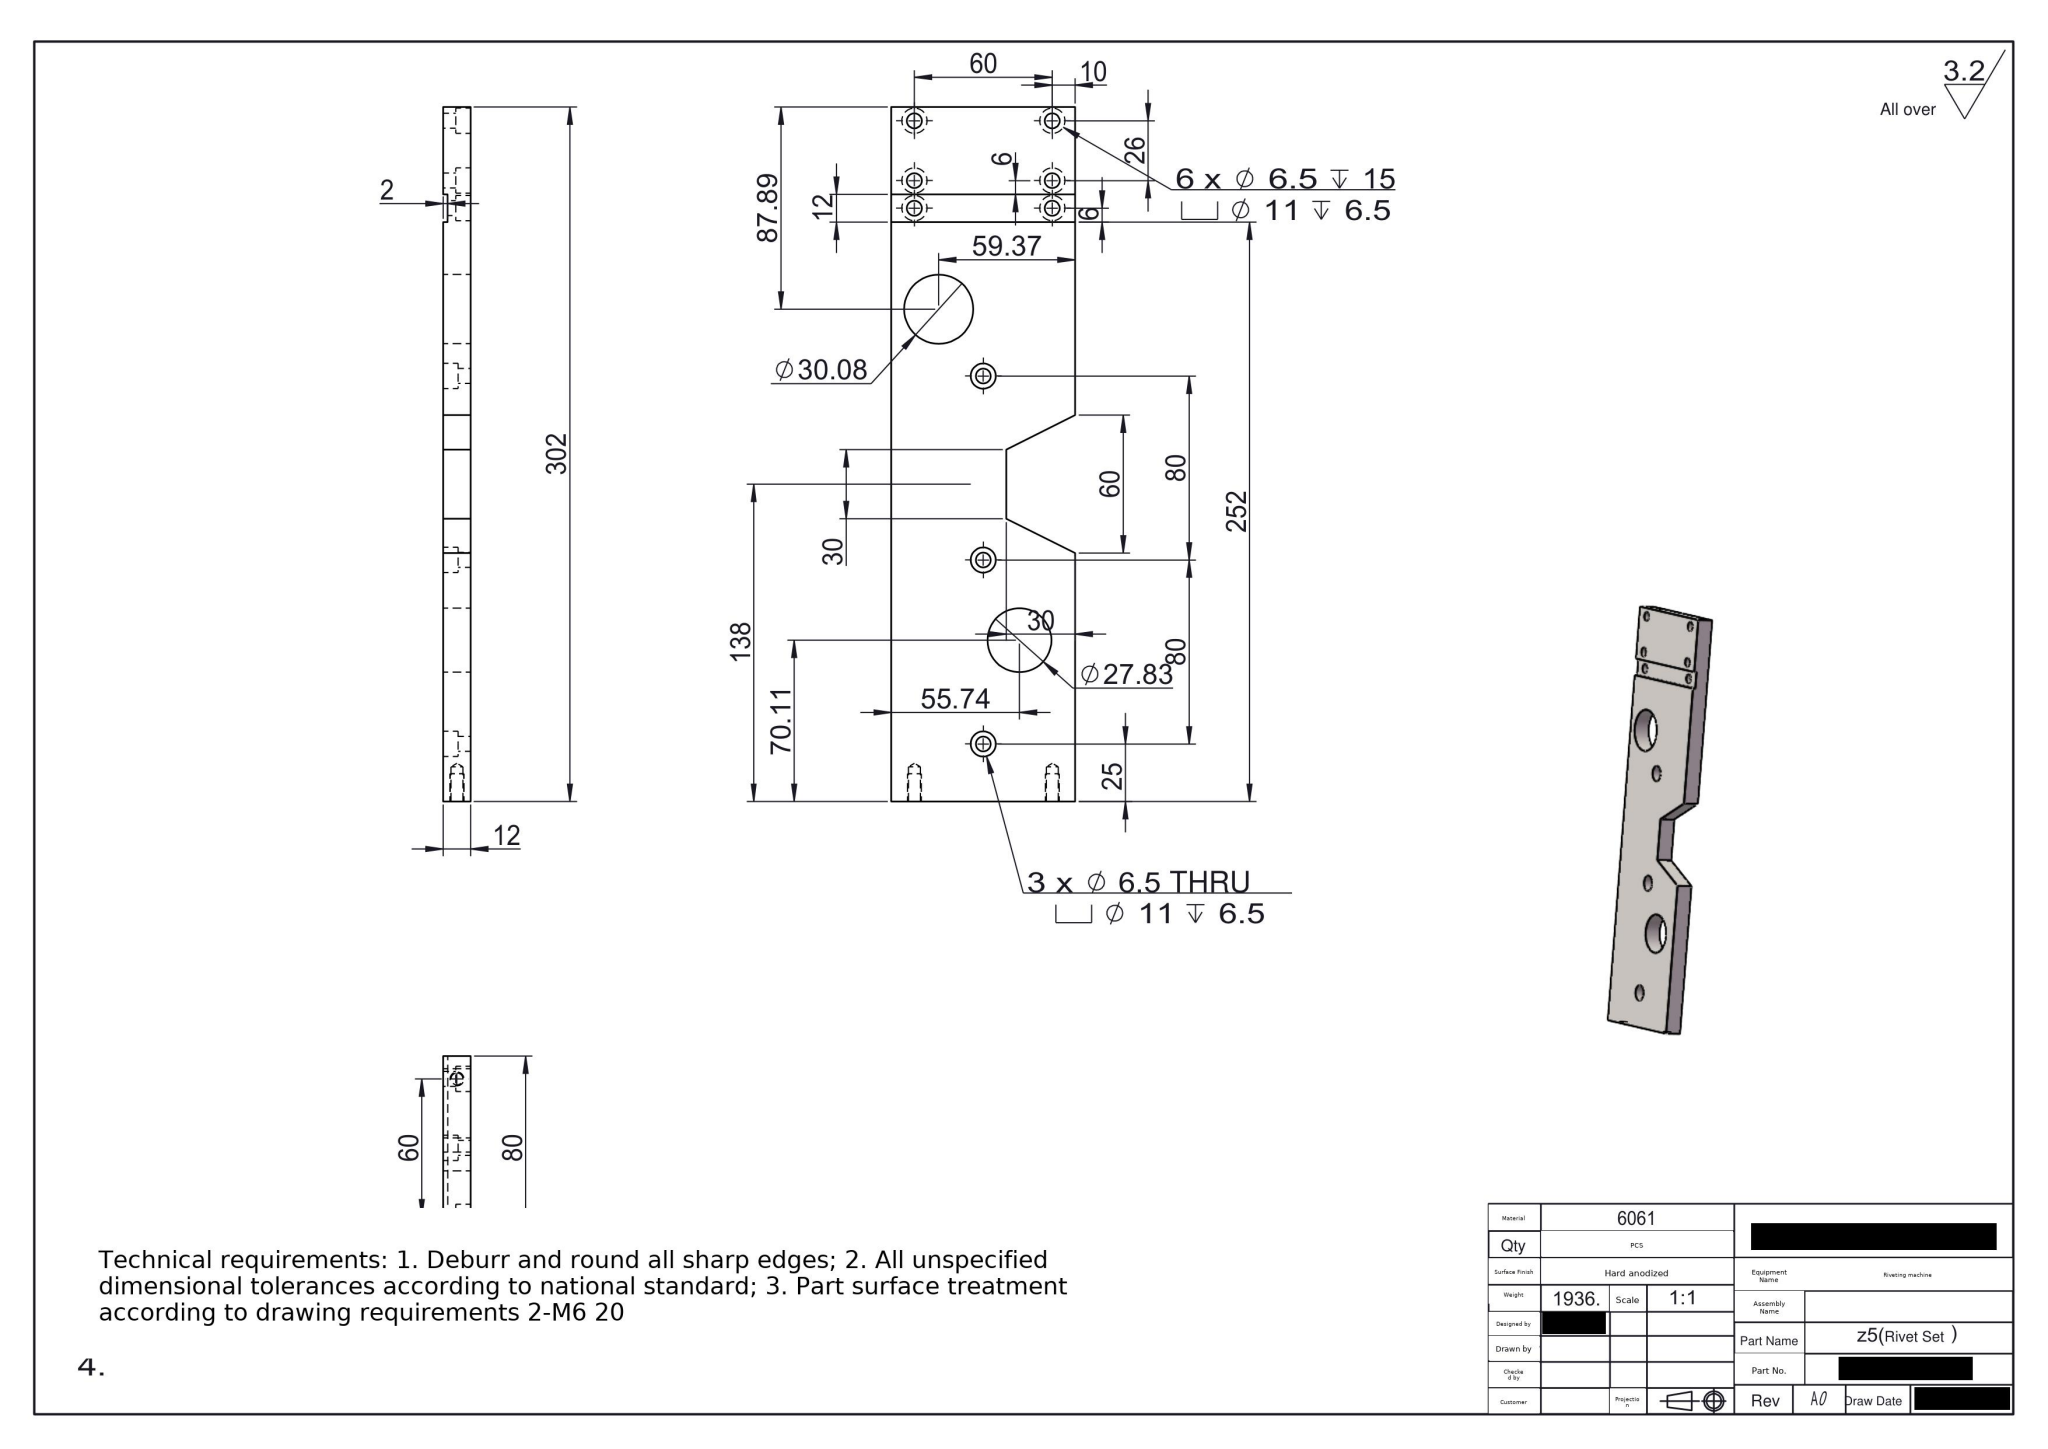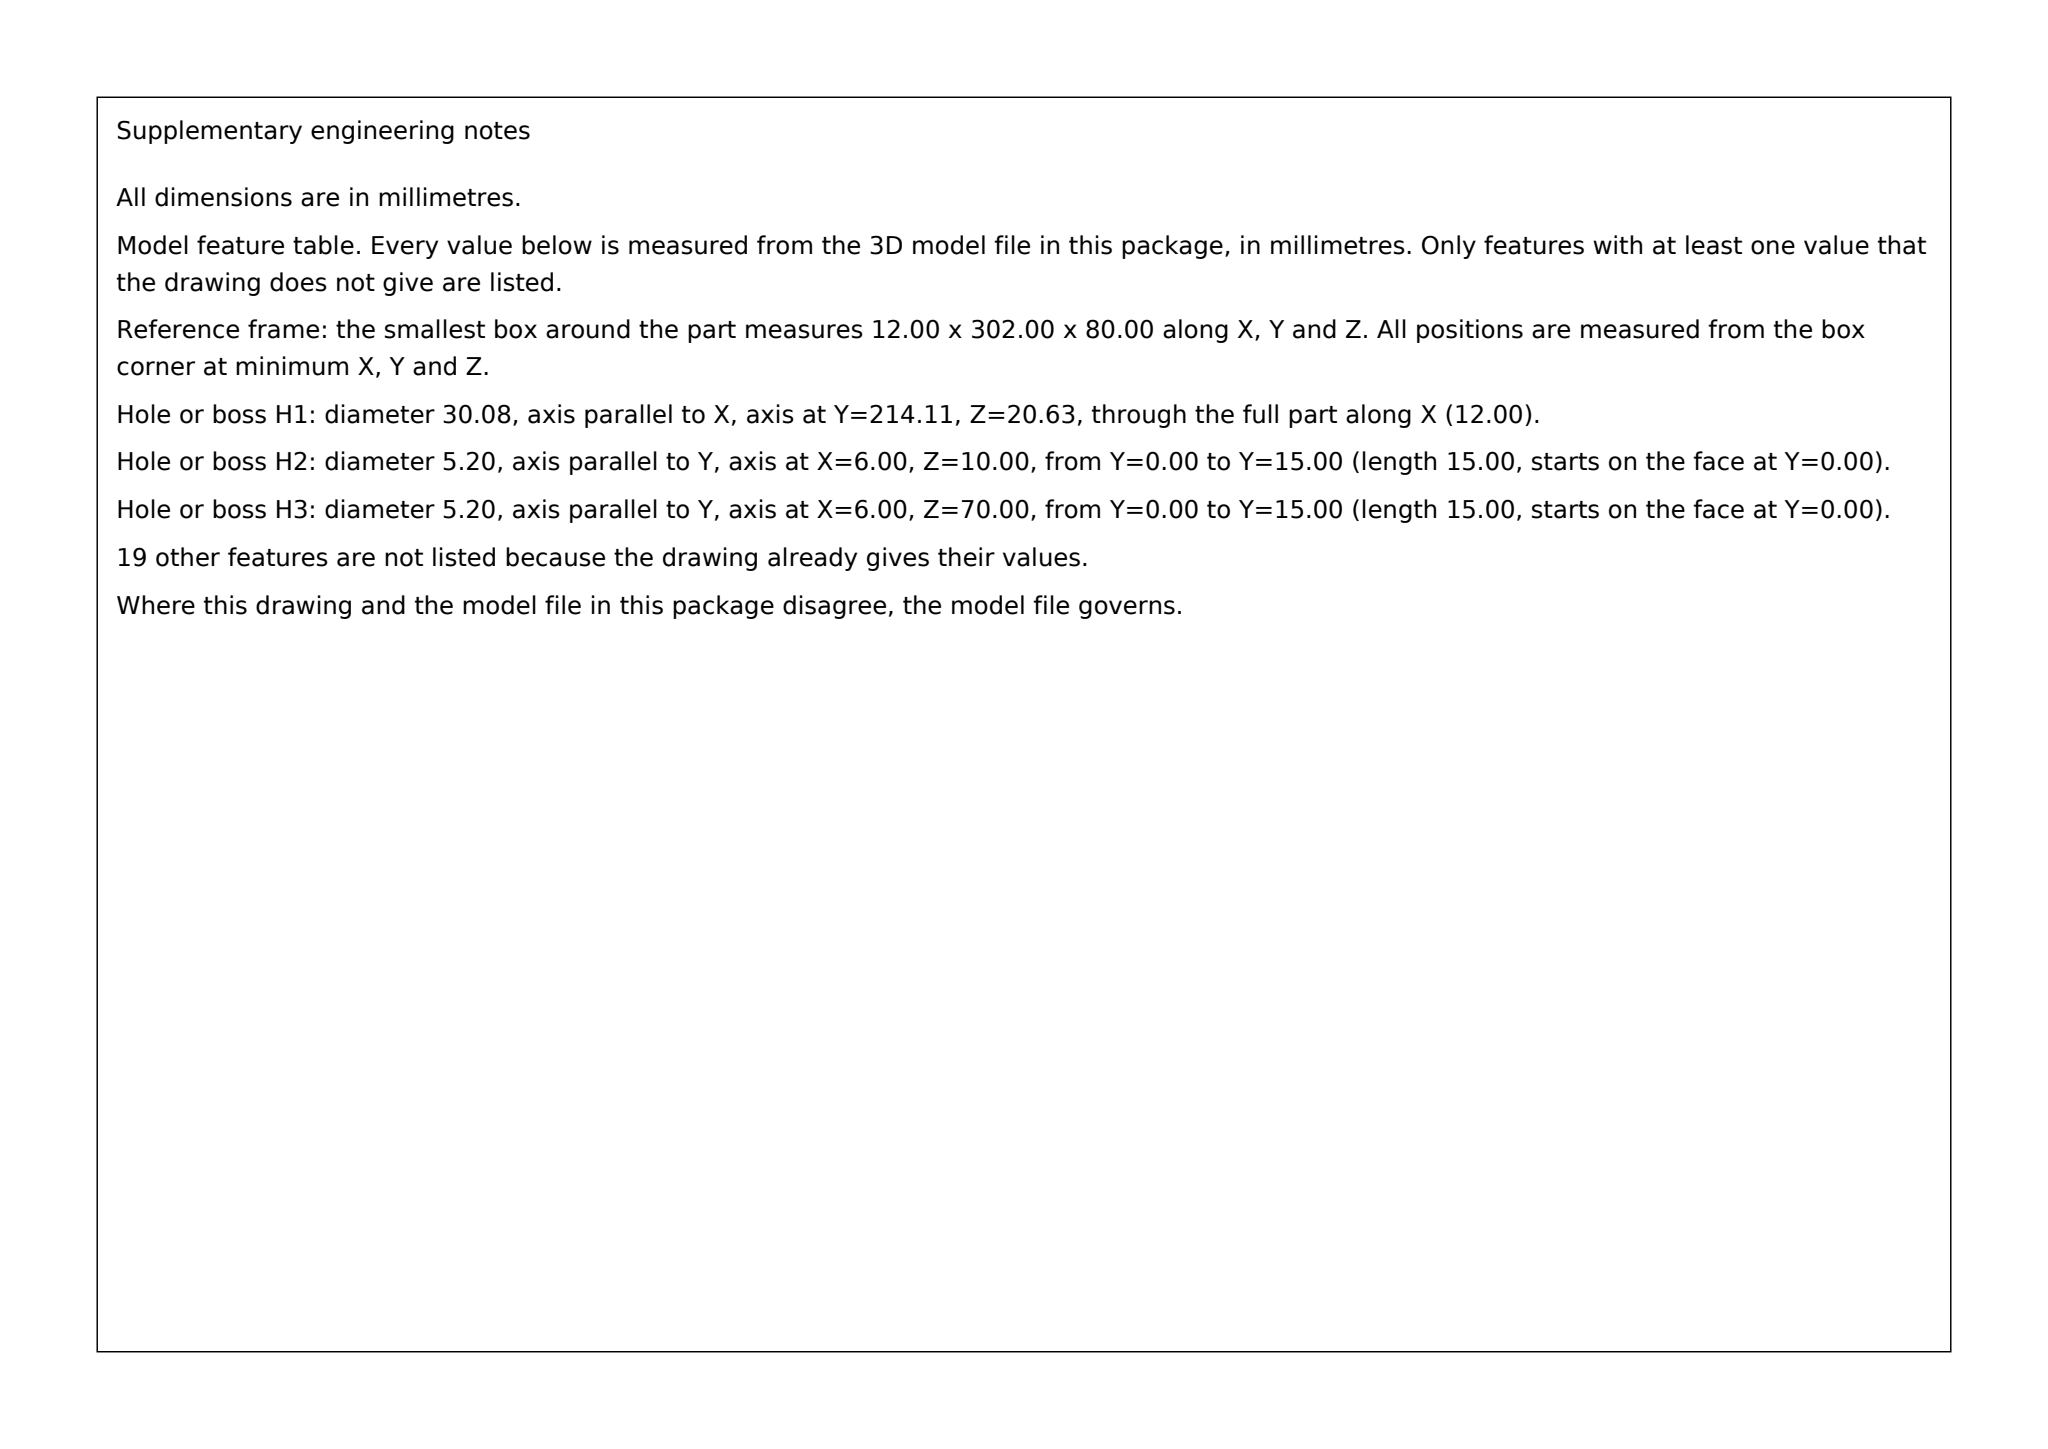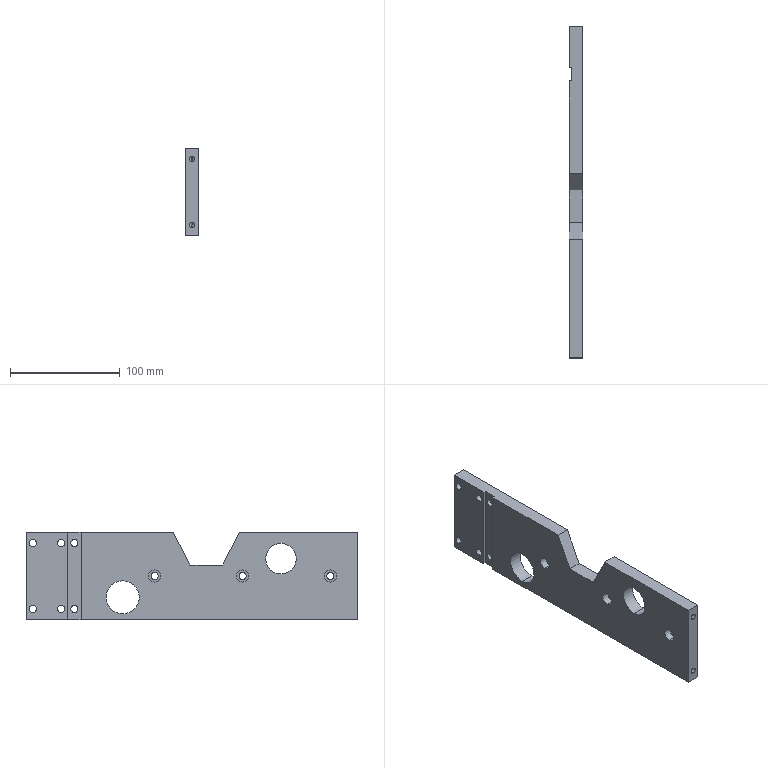Part | SolidWorks | mm | material 6061 | 1 solid | 71 faces | box 12 x 302 x 80 mm | volume 248247 mm3 | cylinder 44 | plane 23 | cone 4 | commonest cylinder face diameters 11 x18 6.5 x18 5.2 x4 30.078 x2 27.827 x2
build123d program:
from build123d import *

# Parameters (mm, degrees)
SKETCH1_W                                           = 12
SKETCH1_H                                           = 302
BOSS_EXTRUDE1_DEPTH                                 = 80
SKETCH3_W                                           = 80
SKETCH3_H                                           = 12
CUT_EXTRUDE1_DEPTH                                  = 2
CYLINDRICAL_COUNTERSUNK_HOLE_FOR_M6_HEX_D           = 6.5
CYLINDRICAL_COUNTERSUNK_HOLE_FOR_M6_HEX_DEPTH       = 15
CYLINDRICAL_COUNTERSUNK_HOLE_FOR_M6_HEX_CBORE_D     = 11
CYLINDRICAL_COUNTERSUNK_HOLE_FOR_M6_HEX_CBORE_DEPTH = 6.5
CYLINDRICAL_COUNTERSUNK_HOLE_FOR_M6_HEX_TIP         = 1.953
CUT_EXTRUDE2_DEPTH                                  = 313.647
M6_TAPPED_HOLE1_D                                   = 5.2
M6_TAPPED_HOLE1_DEPTH                               = 15
M6_TAPPED_HOLE1_TIP                                 = 1.562
CYLINDRICAL_COUNTERSUNK_HOLE_FOR_M6_2_D             = 6.5
CYLINDRICAL_COUNTERSUNK_HOLE_FOR_M6_2_CBORE_D       = 11
CYLINDRICAL_COUNTERSUNK_HOLE_FOR_M6_2_CBORE_DEPTH   = 6.5
SKETCH12_R                                          = 15.039
SKETCH12_R_2                                        = 13.913
CUT_EXTRUDE3_DEPTH                                  = 80


with BuildPart() as part:
    # Sketch1 → Boss-Extrude1 (new body)
    with BuildSketch(Plane.XY):
        with Locations((6, 151)):
            Rectangle(SKETCH1_W, SKETCH1_H)
    extrude(amount=BOSS_EXTRUDE1_DEPTH)

    # Sketch3 → Cut-Extrude1 (cut)
    with BuildSketch(Plane.ZY):
        with Locations((40, 258)):
            Rectangle(SKETCH3_W, SKETCH3_H)
    extrude(amount=-CUT_EXTRUDE1_DEPTH, mode=Mode.SUBTRACT)

    # Cylindrical Countersunk Hole for M6 Hex
    with Locations(Plane(origin=(12, 0, 0), x_dir=(0, 0, -1), z_dir=(1, 0, 0))):
        with Locations((-70, 296), (-10, 296), (-70, 270), (-10, 270), (-10, 258), (-70, 258)):
            CounterBoreHole(CYLINDRICAL_COUNTERSUNK_HOLE_FOR_M6_HEX_D / 2, CYLINDRICAL_COUNTERSUNK_HOLE_FOR_M6_HEX_CBORE_D / 2, CYLINDRICAL_COUNTERSUNK_HOLE_FOR_M6_HEX_CBORE_DEPTH, depth=CYLINDRICAL_COUNTERSUNK_HOLE_FOR_M6_HEX_DEPTH)
            with Locations((0, 0, -(CYLINDRICAL_COUNTERSUNK_HOLE_FOR_M6_HEX_DEPTH + CYLINDRICAL_COUNTERSUNK_HOLE_FOR_M6_HEX_TIP / 2))):  # 118° drill point
                Cone(0, CYLINDRICAL_COUNTERSUNK_HOLE_FOR_M6_HEX_D / 2, CYLINDRICAL_COUNTERSUNK_HOLE_FOR_M6_HEX_TIP, mode=Mode.SUBTRACT)

    # Sketch7 → Cut-Extrude2 (cut, through all)
    with BuildSketch(Plane(origin=(12, 0, 0), x_dir=(0, 0, -1), z_dir=(1, 0, 0))):
        Polygon((-50, 153), (-50, 123), (-80, 108), (-80, 168), align=None)
    extrude(amount=-CUT_EXTRUDE2_DEPTH, mode=Mode.SUBTRACT)

    # M6 Tapped Hole1
    with Locations(Plane(origin=(0, 0, 0), x_dir=(-1, 0, 0), z_dir=(0, -1, 0))):
        with Locations((-6, -10), (-6, -70)):
            Hole(M6_TAPPED_HOLE1_D / 2, depth=M6_TAPPED_HOLE1_DEPTH)
            with Locations((0, 0, -(M6_TAPPED_HOLE1_DEPTH + M6_TAPPED_HOLE1_TIP / 2))):  # 118° drill point
                Cone(0, M6_TAPPED_HOLE1_D / 2, M6_TAPPED_HOLE1_TIP, mode=Mode.SUBTRACT)

    # Cylindrical Countersunk Hole for M6  2 (through all)
    with Locations(Plane.ZY):
        with Locations((40, 25), (40, 105), (40, 185)):
            CounterBoreHole(CYLINDRICAL_COUNTERSUNK_HOLE_FOR_M6_2_D / 2, CYLINDRICAL_COUNTERSUNK_HOLE_FOR_M6_2_CBORE_D / 2, CYLINDRICAL_COUNTERSUNK_HOLE_FOR_M6_2_CBORE_DEPTH)

    # Sketch12 → Cut-Extrude3 (cut)
    with BuildSketch(Plane.ZY):
        with Locations((20.632, 214.112)):
            Circle(SKETCH12_R)
        with Locations((55.743, 70.111)):
            Circle(SKETCH12_R_2)
    extrude(amount=-CUT_EXTRUDE3_DEPTH, mode=Mode.SUBTRACT)


solid = part.part